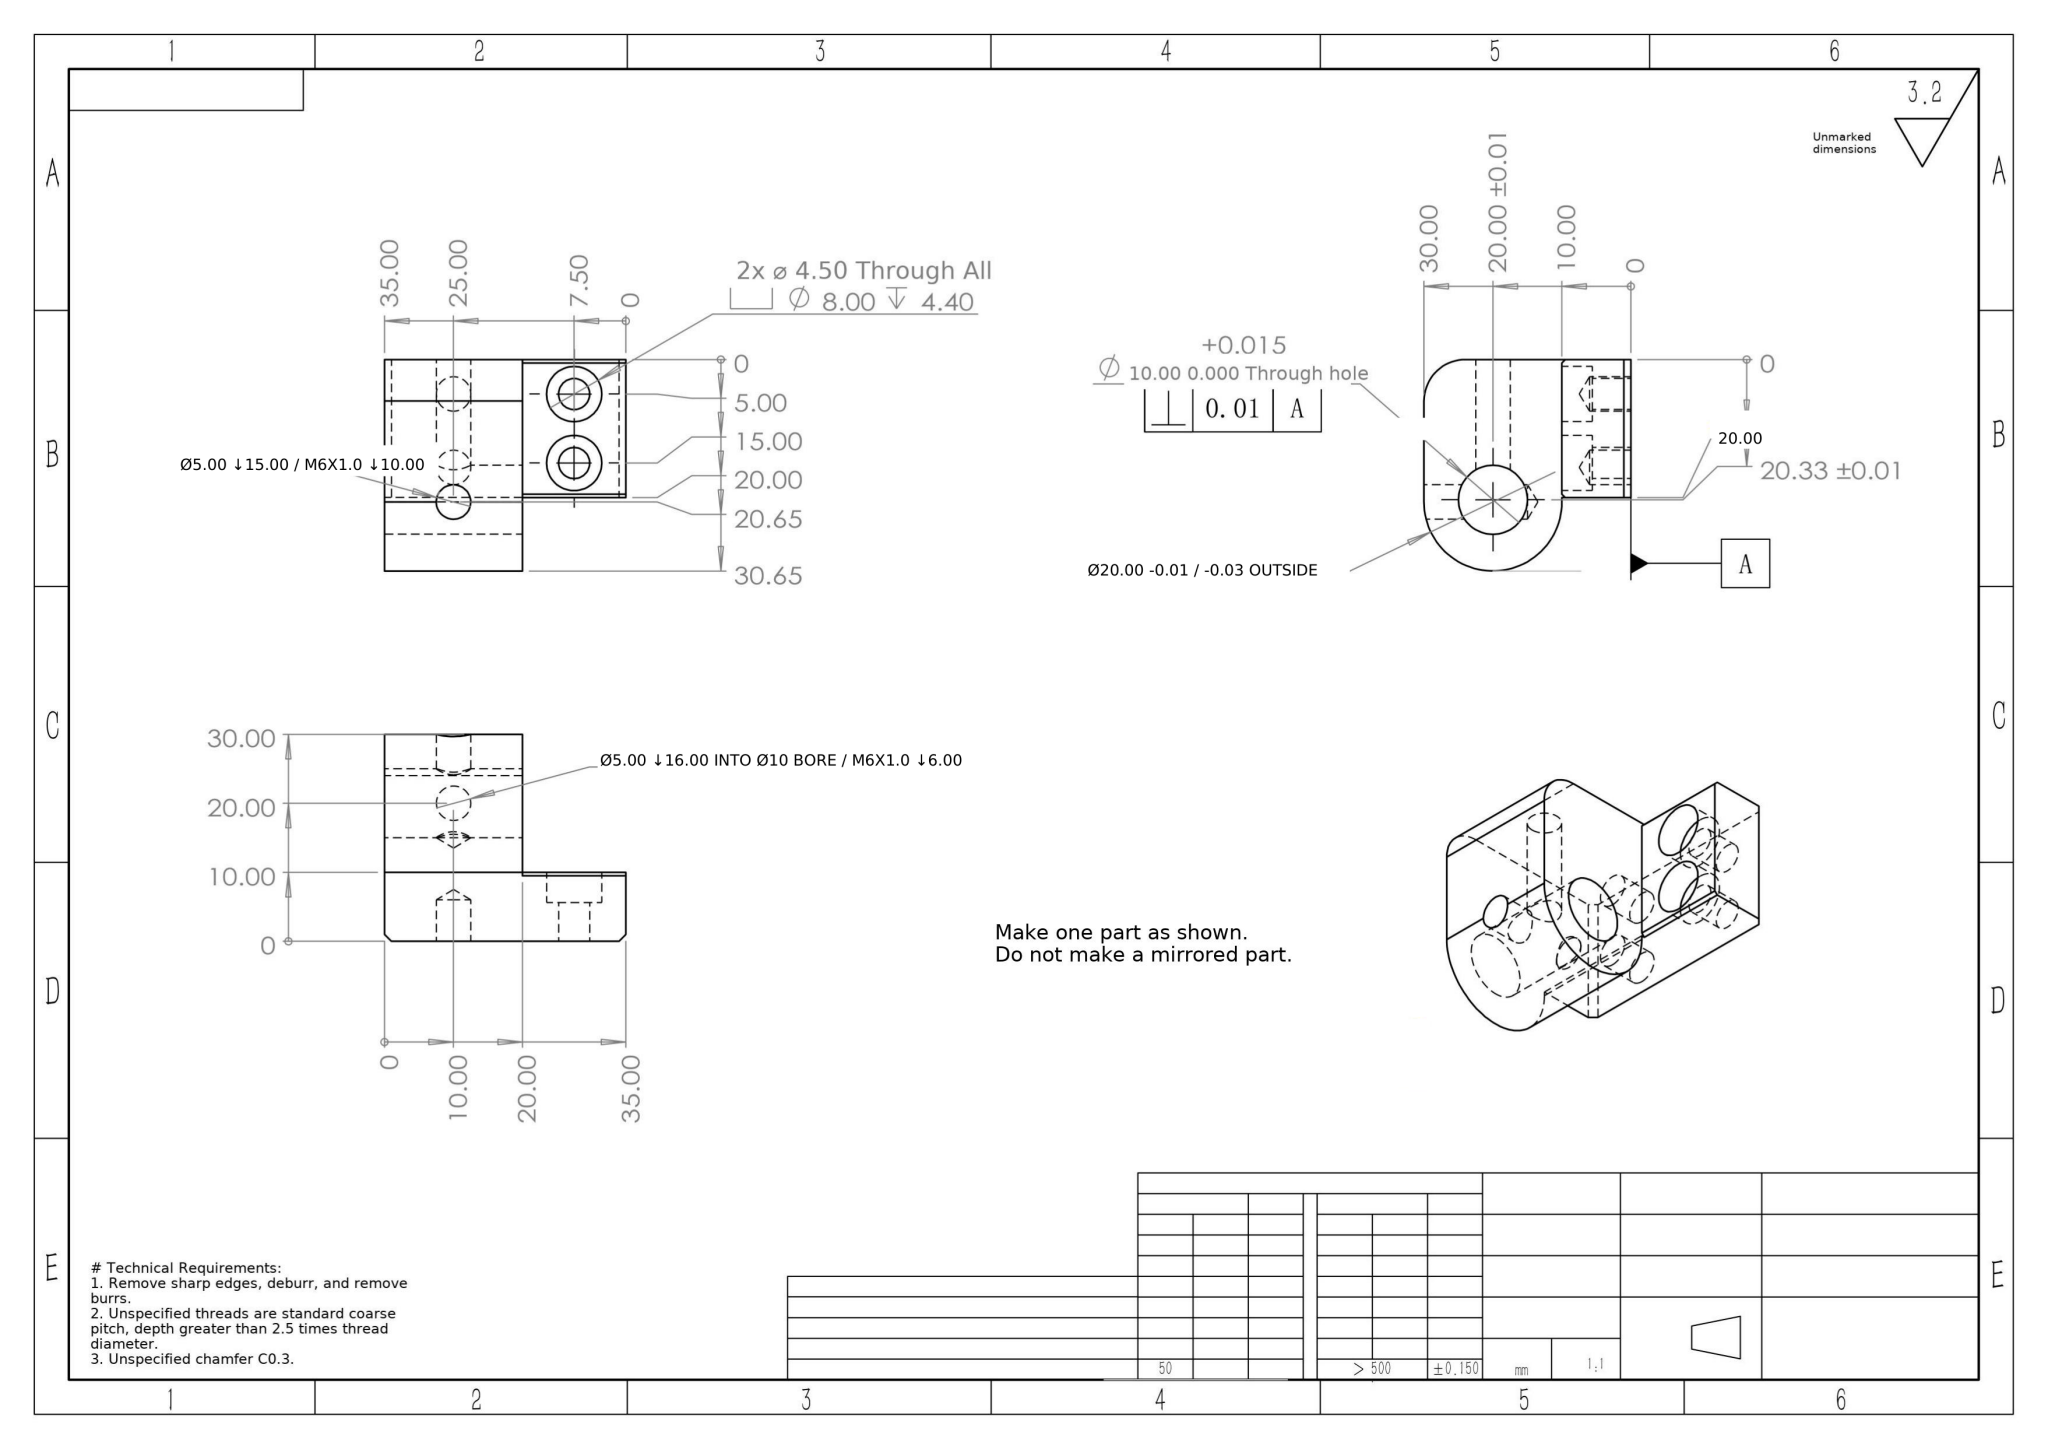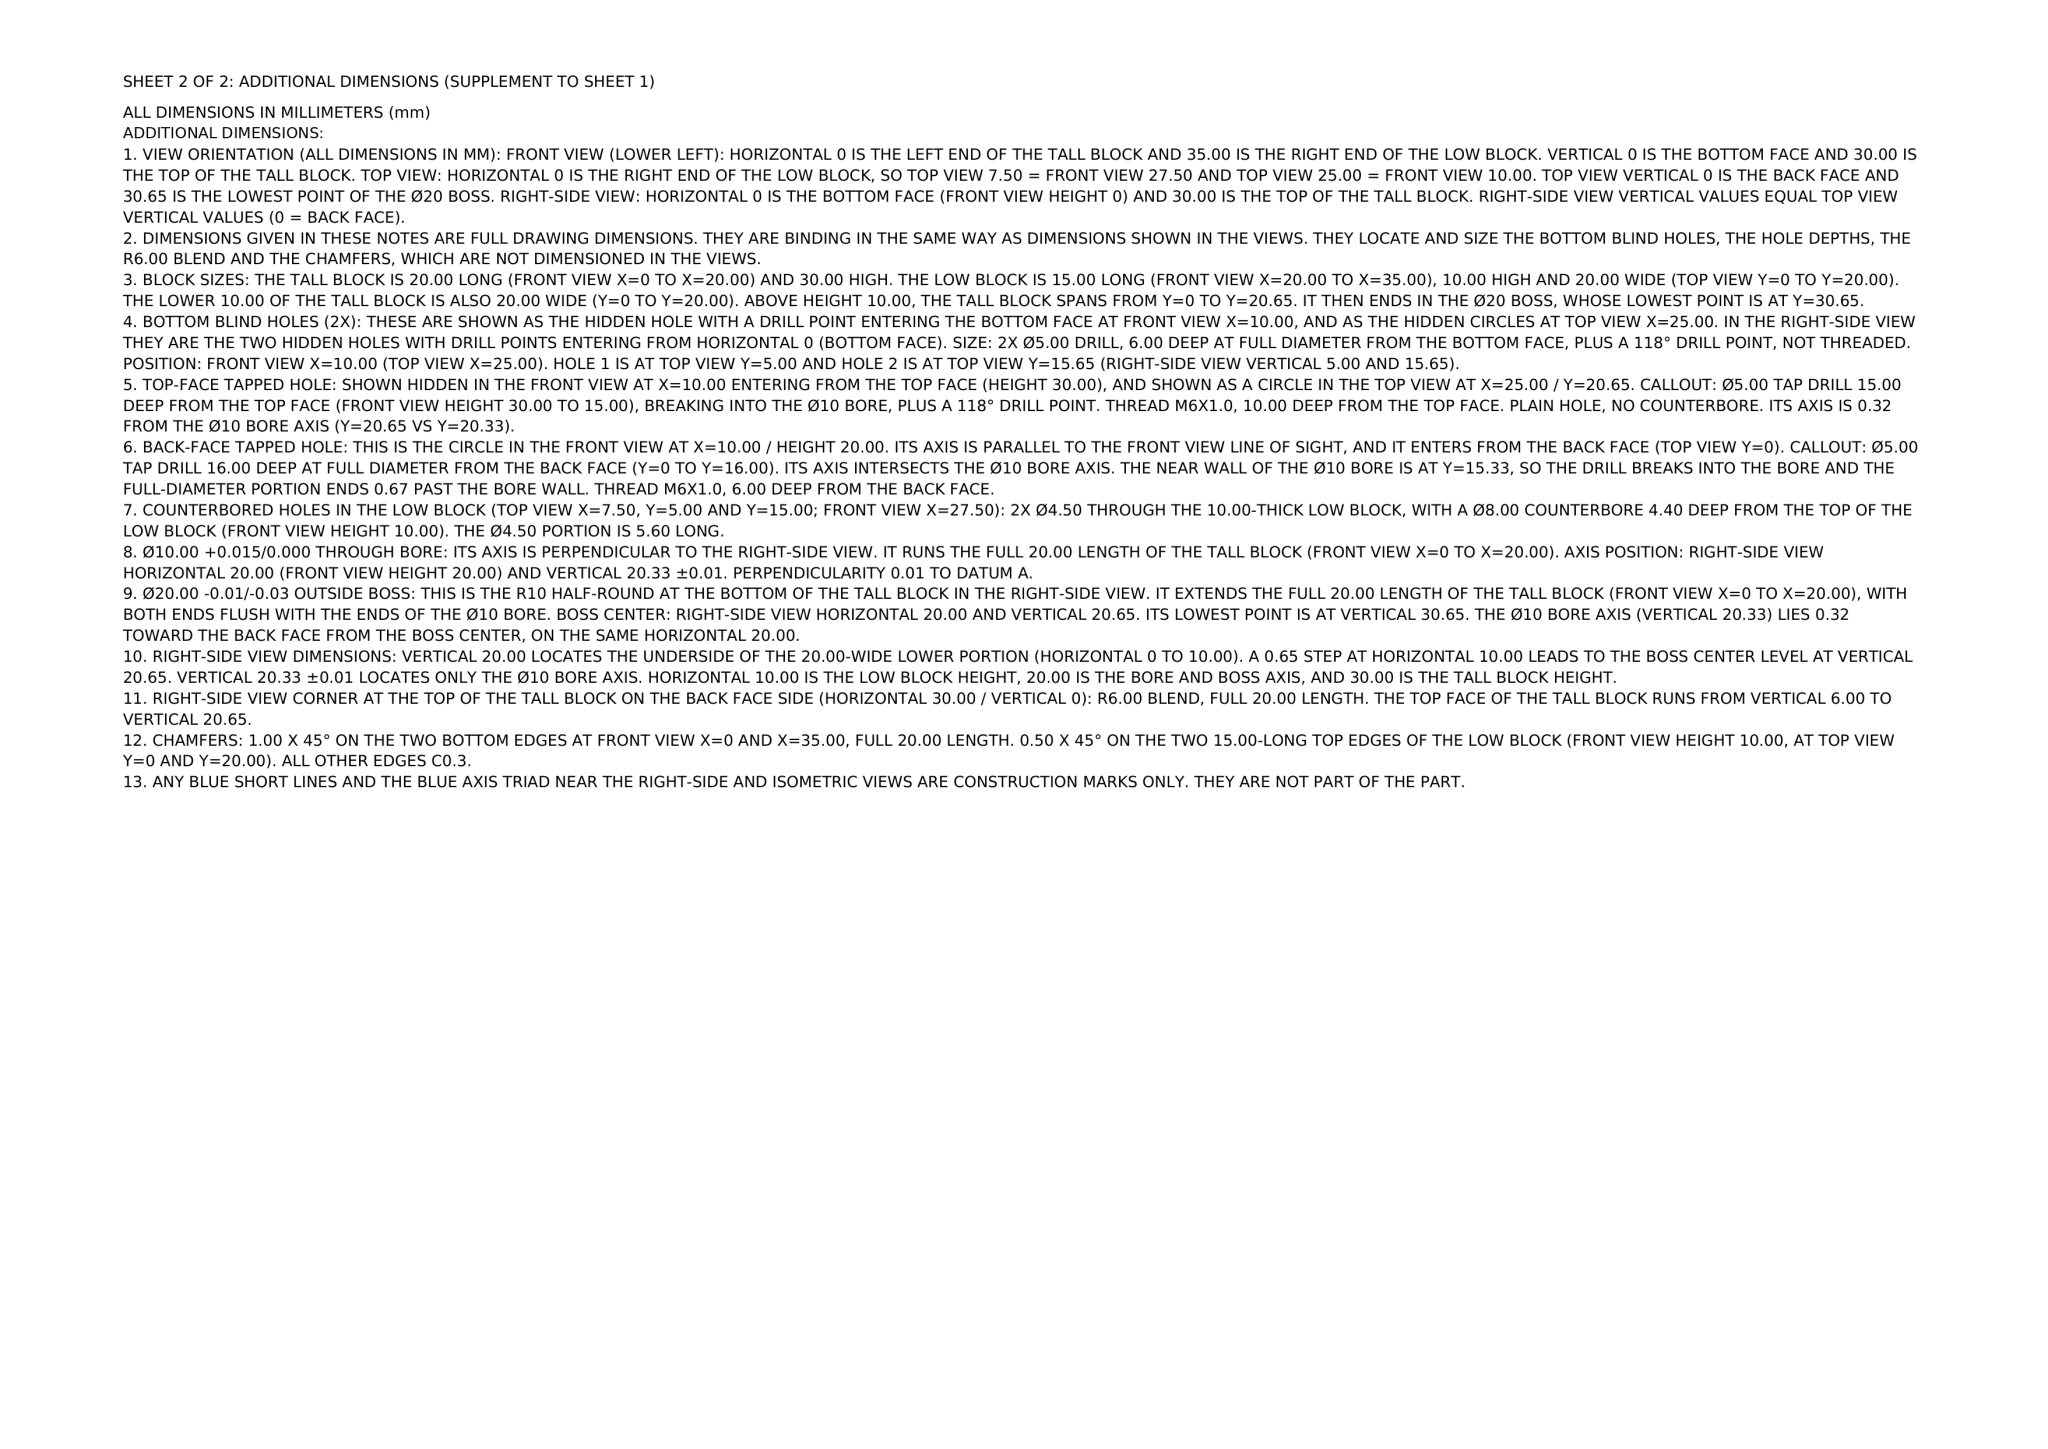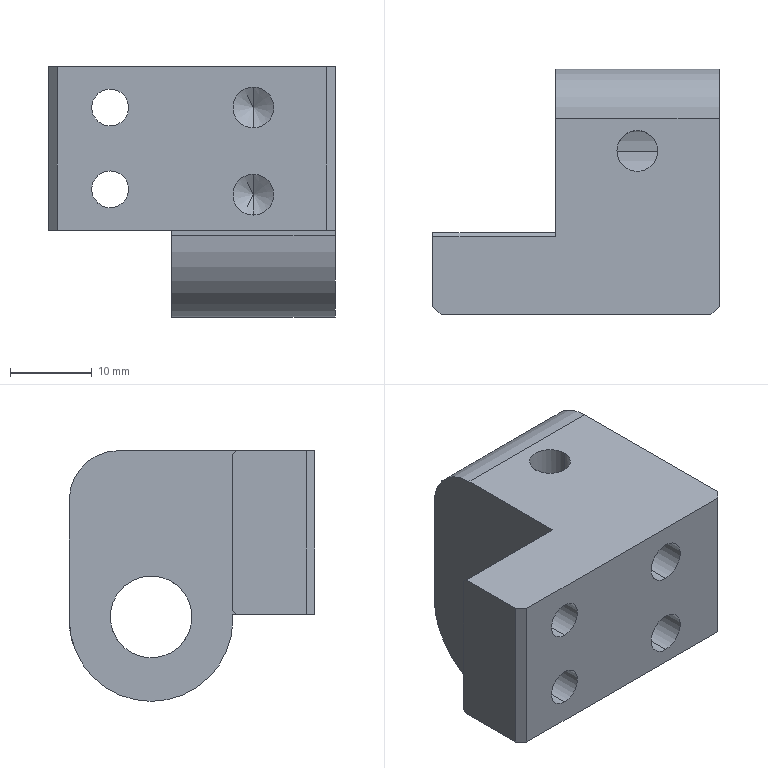Part | NX | mm | 1 solid | 45 faces | box 35 x 30 x 30.65 mm | volume 15359 mm3 | cylinder 24 | plane 15 | cone 6 | commonest cylinder face diameters 5 x11 8 x4 4.5 x4 10 x2 20 x2 12 x1